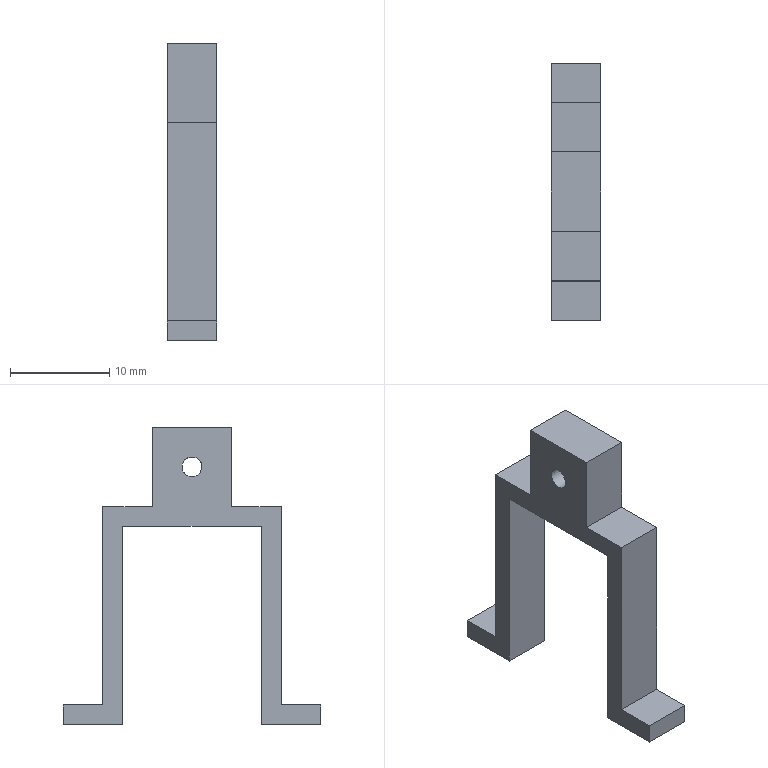Component | NX | TOP_2 | 1 solid | 19 faces | volume 964 mm3 | plane 18 | cylinder 1 | commonest cylinder face diameters 2 x1